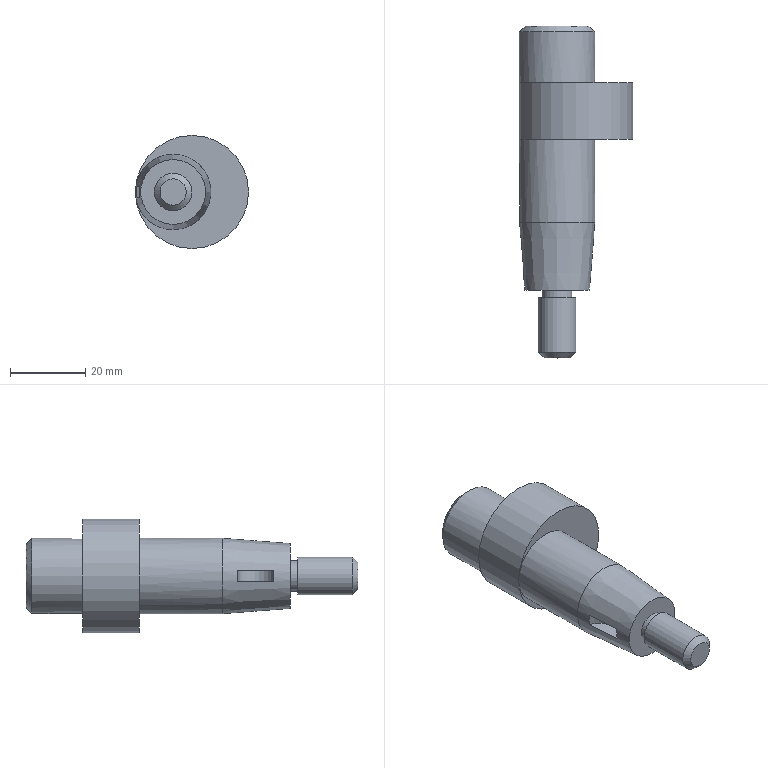Component | NX | ECCENTRIC_SHAFT | 1 solid | 17 faces | box 30 x 88 x 30 mm | volume 28312 mm3 | plane 8 | cylinder 6 | cone 3 | commonest cylinder face diameters 20 x2 10 x2 8 x1 30 x1
STEP:
#1=CARTESIAN_POINT('',(0.,0.,0.));
#2=DIRECTION('',(0.,0.,1.));
#3=DIRECTION('',(1.,0.,0.));
#4=AXIS2_PLACEMENT_3D('',#1,#2,#3);
#5=CARTESIAN_POINT('',(-95.326,-167.11,40.));
#6=VERTEX_POINT('',#5);
#7=CARTESIAN_POINT('',(-95.326,-167.11,50.));
#8=DIRECTION('',(0.,1.,0.));
#9=DIRECTION('',(0.,0.,-1.));
#10=AXIS2_PLACEMENT_3D('',#7,#8,#9);
#11=CIRCLE('',#10,10.);
#12=CARTESIAN_POINT('',(-95.326,-185.11,50.));
#13=DIRECTION('',(0.,1.,0.));
#14=DIRECTION('',(0.,0.,-1.));
#15=AXIS2_PLACEMENT_3D('',#12,#13,#14);
#16=CONICAL_SURFACE('',#15,8.599,0.0777);
#17=CARTESIAN_POINT('',(0.,18.));
#18=DIRECTION('',(1.,0.));
#19=VECTOR('',#18,1.);
#20=LINE('',#17,#19);
#21=(GEOMETRIC_REPRESENTATION_CONTEXT(2)PARAMETRIC_REPRESENTATION_CONTEXT()REPRESENTATION_CONTEXT('',''));
#22=DEFINITIONAL_REPRESENTATION('',(#20),#21);
#23=PCURVE('',#16,#22);
#24=CARTESIAN_POINT('',(-95.326,-203.11,50.));
#25=DIRECTION('',(0.,1.,0.));
#26=DIRECTION('',(0.,0.,-1.));
#27=AXIS2_PLACEMENT_3D('',#24,#25,#26);
#28=CYLINDRICAL_SURFACE('',#27,10.);
#29=CARTESIAN_POINT('',(0.,36.));
#30=DIRECTION('',(1.,0.));
#31=VECTOR('',#30,1.);
#32=LINE('',#29,#31);
#33=(GEOMETRIC_REPRESENTATION_CONTEXT(2)PARAMETRIC_REPRESENTATION_CONTEXT()REPRESENTATION_CONTEXT('',''));
#34=DEFINITIONAL_REPRESENTATION('',(#32),#33);
#35=PCURVE('',#28,#34);
#36=SURFACE_CURVE('',#11,(#23,#35),.PCURVE_S1.);
#37=EDGE_CURVE('',#6,#6,#36,.T.);
#38=ORIENTED_EDGE('',*,*,#37,.F.);
#39=CARTESIAN_POINT('',(-95.326,-185.11,41.401));
#40=VERTEX_POINT('',#39);
#41=CARTESIAN_POINT('',(-95.326,-185.11,41.401));
#42=CARTESIAN_POINT('',(-95.326,-167.11,40.));
#43=B_SPLINE_CURVE_WITH_KNOTS('',1,(#41,#42),.UNSPECIFIED.,.F.,.F.,(2,2),(0.,18.054),.PIECEWISE_BEZIER_KNOTS.);
#44=CARTESIAN_POINT('',(0.,0.));
#45=DIRECTION('',(0.,1.));
#46=VECTOR('',#45,1.);
#47=LINE('',#44,#46);
#48=(GEOMETRIC_REPRESENTATION_CONTEXT(2)PARAMETRIC_REPRESENTATION_CONTEXT()REPRESENTATION_CONTEXT('',''));
#49=DEFINITIONAL_REPRESENTATION('',(#47),#48);
#50=PCURVE('',#16,#49);
#51=CARTESIAN_POINT('',(6.283,0.));
#52=DIRECTION('',(0.,1.));
#53=VECTOR('',#52,1.);
#54=LINE('',#51,#53);
#55=(GEOMETRIC_REPRESENTATION_CONTEXT(2)PARAMETRIC_REPRESENTATION_CONTEXT()REPRESENTATION_CONTEXT('',''));
#56=DEFINITIONAL_REPRESENTATION('',(#54),#55);
#57=PCURVE('',#16,#56);
#58=SEAM_CURVE('',#43,(#50,#57),.PCURVE_S1.);
#59=EDGE_CURVE('',#40,#6,#58,.T.);
#60=ORIENTED_EDGE('',*,*,#59,.F.);
#61=CARTESIAN_POINT('',(-95.326,-185.11,50.));
#62=DIRECTION('',(0.,1.,0.));
#63=DIRECTION('',(0.,0.,-1.));
#64=AXIS2_PLACEMENT_3D('',#61,#62,#63);
#65=CIRCLE('',#64,8.599);
#66=CARTESIAN_POINT('',(0.,0.));
#67=DIRECTION('',(1.,0.));
#68=VECTOR('',#67,1.);
#69=LINE('',#66,#68);
#70=(GEOMETRIC_REPRESENTATION_CONTEXT(2)PARAMETRIC_REPRESENTATION_CONTEXT()REPRESENTATION_CONTEXT('',''));
#71=DEFINITIONAL_REPRESENTATION('',(#69),#70);
#72=PCURVE('',#16,#71);
#73=CARTESIAN_POINT('',(-95.326,-185.11,54.));
#74=DIRECTION('',(0.,1.,0.));
#75=DIRECTION('',(0.,0.,-1.));
#76=AXIS2_PLACEMENT_3D('',#73,#74,#75);
#77=PLANE('',#76);
#78=CARTESIAN_POINT('',(4.,0.));
#79=DIRECTION('',(1.,0.));
#80=AXIS2_PLACEMENT_2D('',#78,#79);
#81=CIRCLE('',#80,8.599);
#82=(GEOMETRIC_REPRESENTATION_CONTEXT(2)PARAMETRIC_REPRESENTATION_CONTEXT()REPRESENTATION_CONTEXT('',''));
#83=DEFINITIONAL_REPRESENTATION('',(#81),#82);
#84=PCURVE('',#77,#83);
#85=SURFACE_CURVE('',#65,(#72,#84),.PCURVE_S1.);
#86=EDGE_CURVE('',#40,#40,#85,.T.);
#87=ORIENTED_EDGE('',*,*,#86,.T.);
#88=ORIENTED_EDGE('',*,*,#59,.T.);
#89=EDGE_LOOP('',(#38,#60,#87,#88));
#90=FACE_BOUND('',#89,.T.);
#91=CARTESIAN_POINT('',(-104.886,-171.267,51.5));
#92=VERTEX_POINT('',#91);
#93=CARTESIAN_POINT('',(-104.142,-180.698,51.5));
#94=VERTEX_POINT('',#93);
#95=CARTESIAN_POINT('',(-104.886,-171.267,51.5));
#96=CARTESIAN_POINT('',(-104.854,-171.674,51.5));
#97=CARTESIAN_POINT('',(-104.822,-172.08,51.5));
#98=CARTESIAN_POINT('',(-104.79,-172.487,51.5));
#99=CARTESIAN_POINT('',(-104.574,-175.224,51.5));
#100=CARTESIAN_POINT('',(-104.358,-177.961,51.5));
#101=CARTESIAN_POINT('',(-104.142,-180.698,51.5));
#102=B_SPLINE_CURVE_WITH_KNOTS('',3,(#95,#96,#97,#98,#99,#100,#101),.UNSPECIFIED.,.F.,.F.,(4,3,4),(0.,0.1293,1.),.UNSPECIFIED.);
#103=CARTESIAN_POINT('',(1.726,13.843));
#104=CARTESIAN_POINT('',(1.739,4.412));
#105=B_SPLINE_CURVE_WITH_KNOTS('',1,(#103,#104),.UNSPECIFIED.,.F.,.F.,(2,2),(0.,1.),.PIECEWISE_BEZIER_KNOTS.);
#106=(GEOMETRIC_REPRESENTATION_CONTEXT(2)PARAMETRIC_REPRESENTATION_CONTEXT()REPRESENTATION_CONTEXT('',''));
#107=DEFINITIONAL_REPRESENTATION('',(#105),#106);
#108=PCURVE('',#16,#107);
#109=CARTESIAN_POINT('',(-106.13,-176.11,51.5));
#110=DIRECTION('',(0.,0.,1.));
#111=DIRECTION('',(-1.,0.,0.));
#112=AXIS2_PLACEMENT_3D('',#109,#110,#111);
#113=PLANE('',#112);
#114=CARTESIAN_POINT('',(-1.244,-4.843));
#115=CARTESIAN_POINT('',(-1.277,-4.436));
#116=CARTESIAN_POINT('',(-1.309,-4.03));
#117=CARTESIAN_POINT('',(-1.341,-3.623));
#118=CARTESIAN_POINT('',(-1.556,-0.8864));
#119=CARTESIAN_POINT('',(-1.772,1.851));
#120=CARTESIAN_POINT('',(-1.988,4.588));
#121=B_SPLINE_CURVE_WITH_KNOTS('',3,(#114,#115,#116,#117,#118,#119,#120),.UNSPECIFIED.,.F.,.F.,(4,3,4),(0.,0.1293,1.),.UNSPECIFIED.);
#122=(GEOMETRIC_REPRESENTATION_CONTEXT(2)PARAMETRIC_REPRESENTATION_CONTEXT()REPRESENTATION_CONTEXT('',''));
#123=DEFINITIONAL_REPRESENTATION('',(#121),#122);
#124=PCURVE('',#113,#123);
#125=SURFACE_CURVE('',#102,(#108,#124),.PCURVE_S1.);
#126=EDGE_CURVE('',#92,#94,#125,.T.);
#127=ORIENTED_EDGE('',*,*,#126,.T.);
#128=CARTESIAN_POINT('',(-104.142,-180.698,48.5));
#129=VERTEX_POINT('',#128);
#130=CARTESIAN_POINT('',(-104.142,-180.698,48.5));
#131=CARTESIAN_POINT('',(-104.306,-180.769,49.496));
#132=CARTESIAN_POINT('',(-104.305,-180.769,50.504));
#133=CARTESIAN_POINT('',(-104.142,-180.698,51.5));
#134=B_SPLINE_CURVE_WITH_KNOTS('',3,(#130,#131,#132,#133),.UNSPECIFIED.,.F.,.F.,(4,4),(0.,1.),.PIECEWISE_BEZIER_KNOTS.);
#135=CARTESIAN_POINT('',(1.402,4.412));
#136=CARTESIAN_POINT('',(1.407,4.409));
#137=CARTESIAN_POINT('',(1.418,4.403));
#138=CARTESIAN_POINT('',(1.433,4.395));
#139=CARTESIAN_POINT('',(1.448,4.387));
#140=CARTESIAN_POINT('',(1.464,4.381));
#141=CARTESIAN_POINT('',(1.479,4.375));
#142=CARTESIAN_POINT('',(1.494,4.37));
#143=CARTESIAN_POINT('',(1.51,4.366));
#144=CARTESIAN_POINT('',(1.525,4.363));
#145=CARTESIAN_POINT('',(1.54,4.361));
#146=CARTESIAN_POINT('',(1.556,4.359));
#147=CARTESIAN_POINT('',(1.571,4.359));
#148=CARTESIAN_POINT('',(1.586,4.359));
#149=CARTESIAN_POINT('',(1.601,4.361));
#150=CARTESIAN_POINT('',(1.617,4.363));
#151=CARTESIAN_POINT('',(1.632,4.366));
#152=CARTESIAN_POINT('',(1.647,4.37));
#153=CARTESIAN_POINT('',(1.663,4.375));
#154=CARTESIAN_POINT('',(1.678,4.381));
#155=CARTESIAN_POINT('',(1.693,4.387));
#156=CARTESIAN_POINT('',(1.709,4.395));
#157=CARTESIAN_POINT('',(1.724,4.403));
#158=CARTESIAN_POINT('',(1.734,4.409));
#159=CARTESIAN_POINT('',(1.739,4.412));
#160=B_SPLINE_CURVE_WITH_KNOTS('',3,(#135,#136,#137,#138,#139,#140,#141,#142,#143,#144,#145,#146,#147,#148,#149,#150,#151,#152,#153,#154,#155,#156,#157,#158,#159),.UNSPECIFIED.,.F.,.F.,(4,1,1,1,1,1,1,1,1,1,1,1,1,1,1,1,1,1,1,1,1,1,4),(0.,0.04545,0.09091,0.1364,0.1818,0.2273,0.2727,0.3182,0.3636,0.4091,0.4545,0.5,0.5455,0.5909,0.6364,0.6818,0.7273,0.7727,0.8182,0.8636,0.9091,0.9545,1.),.QUASI_UNIFORM_KNOTS.);
#161=(GEOMETRIC_REPRESENTATION_CONTEXT(2)PARAMETRIC_REPRESENTATION_CONTEXT()REPRESENTATION_CONTEXT('',''));
#162=DEFINITIONAL_REPRESENTATION('',(#160),#161);
#163=PCURVE('',#16,#162);
#164=CARTESIAN_POINT('',(-106.13,-176.11,51.5));
#165=DIRECTION('',(0.,0.,-1.));
#166=DIRECTION('',(1.,0.,0.));
#167=AXIS2_PLACEMENT_3D('',#164,#165,#166);
#168=CYLINDRICAL_SURFACE('',#167,5.);
#169=CARTESIAN_POINT('',(7.445,3.));
#170=CARTESIAN_POINT('',(7.447,2.955));
#171=CARTESIAN_POINT('',(7.45,2.864));
#172=CARTESIAN_POINT('',(7.454,2.728));
#173=CARTESIAN_POINT('',(7.458,2.592));
#174=CARTESIAN_POINT('',(7.461,2.456));
#175=CARTESIAN_POINT('',(7.464,2.319));
#176=CARTESIAN_POINT('',(7.466,2.183));
#177=CARTESIAN_POINT('',(7.468,2.046));
#178=CARTESIAN_POINT('',(7.47,1.91));
#179=CARTESIAN_POINT('',(7.471,1.773));
#180=CARTESIAN_POINT('',(7.472,1.637));
#181=CARTESIAN_POINT('',(7.472,1.5));
#182=CARTESIAN_POINT('',(7.472,1.363));
#183=CARTESIAN_POINT('',(7.471,1.227));
#184=CARTESIAN_POINT('',(7.47,1.09));
#185=CARTESIAN_POINT('',(7.468,0.9535));
#186=CARTESIAN_POINT('',(7.466,0.817));
#187=CARTESIAN_POINT('',(7.464,0.6806));
#188=CARTESIAN_POINT('',(7.461,0.5442));
#189=CARTESIAN_POINT('',(7.458,0.408));
#190=CARTESIAN_POINT('',(7.454,0.2718));
#191=CARTESIAN_POINT('',(7.45,0.1358));
#192=CARTESIAN_POINT('',(7.447,0.04526));
#193=CARTESIAN_POINT('',(7.445,0.));
#194=B_SPLINE_CURVE_WITH_KNOTS('',3,(#169,#170,#171,#172,#173,#174,#175,#176,#177,#178,#179,#180,#181,#182,#183,#184,#185,#186,#187,#188,#189,#190,#191,#192,#193),.UNSPECIFIED.,.F.,.F.,(4,1,1,1,1,1,1,1,1,1,1,1,1,1,1,1,1,1,1,1,1,1,4),(0.,0.04545,0.09091,0.1364,0.1818,0.2273,0.2727,0.3182,0.3636,0.4091,0.4545,0.5,0.5455,0.5909,0.6364,0.6818,0.7273,0.7727,0.8182,0.8636,0.9091,0.9545,1.),.QUASI_UNIFORM_KNOTS.);
#195=(GEOMETRIC_REPRESENTATION_CONTEXT(2)PARAMETRIC_REPRESENTATION_CONTEXT()REPRESENTATION_CONTEXT('',''));
#196=DEFINITIONAL_REPRESENTATION('',(#194),#195);
#197=PCURVE('',#168,#196);
#198=SURFACE_CURVE('',#134,(#163,#197),.PCURVE_S1.);
#199=EDGE_CURVE('',#129,#94,#198,.T.);
#200=ORIENTED_EDGE('',*,*,#199,.F.);
#201=CARTESIAN_POINT('',(-104.886,-171.267,48.5));
#202=VERTEX_POINT('',#201);
#203=CARTESIAN_POINT('',(-104.886,-171.267,48.5));
#204=CARTESIAN_POINT('',(-104.854,-171.674,48.5));
#205=CARTESIAN_POINT('',(-104.822,-172.08,48.5));
#206=CARTESIAN_POINT('',(-104.79,-172.487,48.5));
#207=CARTESIAN_POINT('',(-104.574,-175.224,48.5));
#208=CARTESIAN_POINT('',(-104.358,-177.961,48.5));
#209=CARTESIAN_POINT('',(-104.142,-180.698,48.5));
#210=B_SPLINE_CURVE_WITH_KNOTS('',3,(#203,#204,#205,#206,#207,#208,#209),.UNSPECIFIED.,.F.,.F.,(4,3,4),(0.,0.1293,1.),.UNSPECIFIED.);
#211=CARTESIAN_POINT('',(1.415,13.843));
#212=CARTESIAN_POINT('',(1.402,4.412));
#213=B_SPLINE_CURVE_WITH_KNOTS('',1,(#211,#212),.UNSPECIFIED.,.F.,.F.,(2,2),(0.,1.),.PIECEWISE_BEZIER_KNOTS.);
#214=(GEOMETRIC_REPRESENTATION_CONTEXT(2)PARAMETRIC_REPRESENTATION_CONTEXT()REPRESENTATION_CONTEXT('',''));
#215=DEFINITIONAL_REPRESENTATION('',(#213),#214);
#216=PCURVE('',#16,#215);
#217=CARTESIAN_POINT('',(-106.13,-176.11,48.5));
#218=DIRECTION('',(0.,0.,1.));
#219=DIRECTION('',(-1.,0.,0.));
#220=AXIS2_PLACEMENT_3D('',#217,#218,#219);
#221=PLANE('',#220);
#222=CARTESIAN_POINT('',(-1.244,-4.843));
#223=CARTESIAN_POINT('',(-1.277,-4.436));
#224=CARTESIAN_POINT('',(-1.309,-4.03));
#225=CARTESIAN_POINT('',(-1.341,-3.623));
#226=CARTESIAN_POINT('',(-1.556,-0.8864));
#227=CARTESIAN_POINT('',(-1.772,1.851));
#228=CARTESIAN_POINT('',(-1.988,4.588));
#229=B_SPLINE_CURVE_WITH_KNOTS('',3,(#222,#223,#224,#225,#226,#227,#228),.UNSPECIFIED.,.F.,.F.,(4,3,4),(0.,0.1293,1.),.UNSPECIFIED.);
#230=(GEOMETRIC_REPRESENTATION_CONTEXT(2)PARAMETRIC_REPRESENTATION_CONTEXT()REPRESENTATION_CONTEXT('',''));
#231=DEFINITIONAL_REPRESENTATION('',(#229),#230);
#232=PCURVE('',#221,#231);
#233=SURFACE_CURVE('',#210,(#216,#232),.PCURVE_S1.);
#234=EDGE_CURVE('',#202,#129,#233,.T.);
#235=ORIENTED_EDGE('',*,*,#234,.F.);
#236=CARTESIAN_POINT('',(-104.886,-171.267,51.5));
#237=CARTESIAN_POINT('',(-105.046,-171.226,50.5));
#238=CARTESIAN_POINT('',(-105.046,-171.226,49.5));
#239=CARTESIAN_POINT('',(-104.886,-171.267,48.5));
#240=B_SPLINE_CURVE_WITH_KNOTS('',3,(#236,#237,#238,#239),.UNSPECIFIED.,.F.,.F.,(4,4),(0.,1.),.PIECEWISE_BEZIER_KNOTS.);
#241=CARTESIAN_POINT('',(1.726,13.843));
#242=CARTESIAN_POINT('',(1.415,13.843));
#243=B_SPLINE_CURVE_WITH_KNOTS('',1,(#241,#242),.UNSPECIFIED.,.F.,.F.,(2,2),(0.,1.),.PIECEWISE_BEZIER_KNOTS.);
#244=(GEOMETRIC_REPRESENTATION_CONTEXT(2)PARAMETRIC_REPRESENTATION_CONTEXT()REPRESENTATION_CONTEXT('',''));
#245=DEFINITIONAL_REPRESENTATION('',(#243),#244);
#246=PCURVE('',#16,#245);
#247=CARTESIAN_POINT('',(4.964,0.));
#248=CARTESIAN_POINT('',(4.962,0.04545));
#249=CARTESIAN_POINT('',(4.96,0.1364));
#250=CARTESIAN_POINT('',(4.956,0.2727));
#251=CARTESIAN_POINT('',(4.952,0.4091));
#252=CARTESIAN_POINT('',(4.949,0.5455));
#253=CARTESIAN_POINT('',(4.946,0.6818));
#254=CARTESIAN_POINT('',(4.944,0.8182));
#255=CARTESIAN_POINT('',(4.942,0.9545));
#256=CARTESIAN_POINT('',(4.941,1.091));
#257=CARTESIAN_POINT('',(4.94,1.227));
#258=CARTESIAN_POINT('',(4.939,1.364));
#259=CARTESIAN_POINT('',(4.939,1.5));
#260=CARTESIAN_POINT('',(4.939,1.636));
#261=CARTESIAN_POINT('',(4.94,1.773));
#262=CARTESIAN_POINT('',(4.941,1.909));
#263=CARTESIAN_POINT('',(4.942,2.045));
#264=CARTESIAN_POINT('',(4.944,2.182));
#265=CARTESIAN_POINT('',(4.946,2.318));
#266=CARTESIAN_POINT('',(4.949,2.455));
#267=CARTESIAN_POINT('',(4.952,2.591));
#268=CARTESIAN_POINT('',(4.956,2.727));
#269=CARTESIAN_POINT('',(4.96,2.864));
#270=CARTESIAN_POINT('',(4.962,2.955));
#271=CARTESIAN_POINT('',(4.964,3.));
#272=B_SPLINE_CURVE_WITH_KNOTS('',3,(#247,#248,#249,#250,#251,#252,#253,#254,#255,#256,#257,#258,#259,#260,#261,#262,#263,#264,#265,#266,#267,#268,#269,#270,#271),.UNSPECIFIED.,.F.,.F.,(4,1,1,1,1,1,1,1,1,1,1,1,1,1,1,1,1,1,1,1,1,1,4),(0.,0.04545,0.09091,0.1364,0.1818,0.2273,0.2727,0.3182,0.3636,0.4091,0.4545,0.5,0.5455,0.5909,0.6364,0.6818,0.7273,0.7727,0.8182,0.8636,0.9091,0.9545,1.),.QUASI_UNIFORM_KNOTS.);
#273=(GEOMETRIC_REPRESENTATION_CONTEXT(2)PARAMETRIC_REPRESENTATION_CONTEXT()REPRESENTATION_CONTEXT('',''));
#274=DEFINITIONAL_REPRESENTATION('',(#272),#273);
#275=PCURVE('',#168,#274);
#276=SURFACE_CURVE('',#240,(#246,#275),.PCURVE_S1.);
#277=EDGE_CURVE('',#92,#202,#276,.T.);
#278=ORIENTED_EDGE('',*,*,#277,.F.);
#279=EDGE_LOOP('',(#127,#200,#235,#278));
#280=FACE_BOUND('',#279,.T.);
#281=ADVANCED_FACE('',(#90,#280),#16,.T.);
#282=ORIENTED_EDGE('',*,*,#37,.T.);
#283=CARTESIAN_POINT('',(-95.326,-145.11,40.));
#284=VERTEX_POINT('',#283);
#285=CARTESIAN_POINT('',(-95.326,-167.11,40.));
#286=CARTESIAN_POINT('',(-95.326,-145.11,40.));
#287=B_SPLINE_CURVE_WITH_KNOTS('',1,(#285,#286),.UNSPECIFIED.,.F.,.F.,(2,2),(36.,58.),.PIECEWISE_BEZIER_KNOTS.);
#288=CARTESIAN_POINT('',(6.283,0.));
#289=DIRECTION('',(0.,1.));
#290=VECTOR('',#289,1.);
#291=LINE('',#288,#290);
#292=(GEOMETRIC_REPRESENTATION_CONTEXT(2)PARAMETRIC_REPRESENTATION_CONTEXT()REPRESENTATION_CONTEXT('',''));
#293=DEFINITIONAL_REPRESENTATION('',(#291),#292);
#294=PCURVE('',#28,#293);
#295=CARTESIAN_POINT('',(0.,0.));
#296=DIRECTION('',(0.,1.));
#297=VECTOR('',#296,1.);
#298=LINE('',#295,#297);
#299=(GEOMETRIC_REPRESENTATION_CONTEXT(2)PARAMETRIC_REPRESENTATION_CONTEXT()REPRESENTATION_CONTEXT('',''));
#300=DEFINITIONAL_REPRESENTATION('',(#298),#299);
#301=PCURVE('',#28,#300);
#302=SEAM_CURVE('',#287,(#294,#301),.PCURVE_S1.);
#303=EDGE_CURVE('',#6,#284,#302,.T.);
#304=ORIENTED_EDGE('',*,*,#303,.T.);
#305=CARTESIAN_POINT('',(-105.326,-145.11,50.));
#306=VERTEX_POINT('',#305);
#307=CARTESIAN_POINT('',(-95.326,-145.11,50.));
#308=DIRECTION('',(0.,1.,0.));
#309=DIRECTION('',(0.,0.,-1.));
#310=AXIS2_PLACEMENT_3D('',#307,#308,#309);
#311=CIRCLE('',#310,10.);
#312=CARTESIAN_POINT('',(0.,58.));
#313=DIRECTION('',(1.,0.));
#314=VECTOR('',#313,1.);
#315=LINE('',#312,#314);
#316=(GEOMETRIC_REPRESENTATION_CONTEXT(2)PARAMETRIC_REPRESENTATION_CONTEXT()REPRESENTATION_CONTEXT('',''));
#317=DEFINITIONAL_REPRESENTATION('',(#315),#316);
#318=PCURVE('',#28,#317);
#319=CARTESIAN_POINT('',(-90.326,-145.11,50.));
#320=DIRECTION('',(0.,1.,0.));
#321=DIRECTION('',(0.,0.,-1.));
#322=AXIS2_PLACEMENT_3D('',#319,#320,#321);
#323=PLANE('',#322);
#324=CARTESIAN_POINT('',(0.,5.));
#325=DIRECTION('',(1.,0.));
#326=AXIS2_PLACEMENT_2D('',#324,#325);
#327=CIRCLE('',#326,10.);
#328=(GEOMETRIC_REPRESENTATION_CONTEXT(2)PARAMETRIC_REPRESENTATION_CONTEXT()REPRESENTATION_CONTEXT('',''));
#329=DEFINITIONAL_REPRESENTATION('',(#327),#328);
#330=PCURVE('',#323,#329);
#331=SURFACE_CURVE('',#311,(#318,#330),.PCURVE_S1.);
#332=EDGE_CURVE('',#306,#284,#331,.T.);
#333=ORIENTED_EDGE('',*,*,#332,.F.);
#334=CARTESIAN_POINT('',(-95.326,-145.11,50.));
#335=DIRECTION('',(0.,1.,0.));
#336=DIRECTION('',(0.,0.,-1.));
#337=AXIS2_PLACEMENT_3D('',#334,#335,#336);
#338=CIRCLE('',#337,10.);
#339=CARTESIAN_POINT('',(-6.283,58.));
#340=DIRECTION('',(1.,0.));
#341=VECTOR('',#340,1.);
#342=LINE('',#339,#341);
#343=(GEOMETRIC_REPRESENTATION_CONTEXT(2)PARAMETRIC_REPRESENTATION_CONTEXT()REPRESENTATION_CONTEXT('',''));
#344=DEFINITIONAL_REPRESENTATION('',(#342),#343);
#345=PCURVE('',#28,#344);
#346=CARTESIAN_POINT('',(0.,5.));
#347=DIRECTION('',(1.,0.));
#348=AXIS2_PLACEMENT_2D('',#346,#347);
#349=CIRCLE('',#348,10.);
#350=(GEOMETRIC_REPRESENTATION_CONTEXT(2)PARAMETRIC_REPRESENTATION_CONTEXT()REPRESENTATION_CONTEXT('',''));
#351=DEFINITIONAL_REPRESENTATION('',(#349),#350);
#352=PCURVE('',#323,#351);
#353=SURFACE_CURVE('',#338,(#345,#352),.PCURVE_S1.);
#354=EDGE_CURVE('',#284,#306,#353,.T.);
#355=ORIENTED_EDGE('',*,*,#354,.F.);
#356=ORIENTED_EDGE('',*,*,#303,.F.);
#357=EDGE_LOOP('',(#282,#304,#333,#355,#356));
#358=FACE_BOUND('',#357,.T.);
#359=ADVANCED_FACE('',(#358),#28,.T.);
#360=CARTESIAN_POINT('',(-95.326,-203.11,46.5));
#361=VERTEX_POINT('',#360);
#362=CARTESIAN_POINT('',(-95.326,-203.11,50.));
#363=DIRECTION('',(0.,-1.,0.));
#364=DIRECTION('',(0.,0.,-1.));
#365=AXIS2_PLACEMENT_3D('',#362,#363,#364);
#366=CIRCLE('',#365,3.5);
#367=CARTESIAN_POINT('',(-95.326,-203.11,50.));
#368=DIRECTION('',(0.,1.,0.));
#369=DIRECTION('',(0.,0.,-1.));
#370=AXIS2_PLACEMENT_3D('',#367,#368,#369);
#371=PLANE('',#370);
#372=CARTESIAN_POINT('',(3.5,0.));
#373=CARTESIAN_POINT('',(3.5,-6.062));
#374=CARTESIAN_POINT('',(-1.75,-3.031));
#375=CARTESIAN_POINT('',(-7.,-0.));
#376=CARTESIAN_POINT('',(-1.75,3.031));
#377=CARTESIAN_POINT('',(3.5,6.062));
#378=CARTESIAN_POINT('',(3.5,0.));
#379=(BOUNDED_CURVE()B_SPLINE_CURVE(2,(#372,#373,#374,#375,#376,#377,#378),.UNSPECIFIED.,.T.,.F.)B_SPLINE_CURVE_WITH_KNOTS((1,2,2,2,2,1),(-2.094,0.,2.094,4.189,6.283,8.378),.UNSPECIFIED.)CURVE()GEOMETRIC_REPRESENTATION_ITEM()RATIONAL_B_SPLINE_CURVE((1.,0.5,1.,0.5,1.,0.5,1.))REPRESENTATION_ITEM(''));
#380=(GEOMETRIC_REPRESENTATION_CONTEXT(2)PARAMETRIC_REPRESENTATION_CONTEXT()REPRESENTATION_CONTEXT('',''));
#381=DEFINITIONAL_REPRESENTATION('',(#379),#380);
#382=PCURVE('',#371,#381);
#383=CARTESIAN_POINT('',(-95.326,-201.61,50.));
#384=DIRECTION('',(0.,1.,0.));
#385=DIRECTION('',(0.,0.,-1.));
#386=AXIS2_PLACEMENT_3D('',#383,#384,#385);
#387=CONICAL_SURFACE('',#386,5.,0.7854);
#388=CARTESIAN_POINT('',(6.283,-1.5));
#389=DIRECTION('',(-1.,0.));
#390=VECTOR('',#389,1.);
#391=LINE('',#388,#390);
#392=(GEOMETRIC_REPRESENTATION_CONTEXT(2)PARAMETRIC_REPRESENTATION_CONTEXT()REPRESENTATION_CONTEXT('',''));
#393=DEFINITIONAL_REPRESENTATION('',(#391),#392);
#394=PCURVE('',#387,#393);
#395=SURFACE_CURVE('',#366,(#382,#394),.PCURVE_S1.);
#396=EDGE_CURVE('',#361,#361,#395,.T.);
#397=ORIENTED_EDGE('',*,*,#396,.T.);
#398=EDGE_LOOP('',(#397));
#399=FACE_BOUND('',#398,.T.);
#400=ADVANCED_FACE('',(#399),#371,.F.);
#401=CARTESIAN_POINT('',(-95.326,-201.61,45.));
#402=VERTEX_POINT('',#401);
#403=CARTESIAN_POINT('',(-95.326,-201.61,50.));
#404=DIRECTION('',(0.,1.,0.));
#405=DIRECTION('',(0.,0.,-1.));
#406=AXIS2_PLACEMENT_3D('',#403,#404,#405);
#407=CIRCLE('',#406,5.);
#408=CARTESIAN_POINT('',(-95.326,-203.11,50.));
#409=DIRECTION('',(0.,1.,0.));
#410=DIRECTION('',(0.,0.,-1.));
#411=AXIS2_PLACEMENT_3D('',#408,#409,#410);
#412=CYLINDRICAL_SURFACE('',#411,5.);
#413=CARTESIAN_POINT('',(0.,1.5));
#414=DIRECTION('',(1.,0.));
#415=VECTOR('',#414,1.);
#416=LINE('',#413,#415);
#417=(GEOMETRIC_REPRESENTATION_CONTEXT(2)PARAMETRIC_REPRESENTATION_CONTEXT()REPRESENTATION_CONTEXT('',''));
#418=DEFINITIONAL_REPRESENTATION('',(#416),#417);
#419=PCURVE('',#412,#418);
#420=CARTESIAN_POINT('',(0.,0.));
#421=DIRECTION('',(1.,0.));
#422=VECTOR('',#421,1.);
#423=LINE('',#420,#422);
#424=(GEOMETRIC_REPRESENTATION_CONTEXT(2)PARAMETRIC_REPRESENTATION_CONTEXT()REPRESENTATION_CONTEXT('',''));
#425=DEFINITIONAL_REPRESENTATION('',(#423),#424);
#426=PCURVE('',#387,#425);
#427=SURFACE_CURVE('',#407,(#419,#426),.PCURVE_S1.);
#428=EDGE_CURVE('',#402,#402,#427,.T.);
#429=ORIENTED_EDGE('',*,*,#428,.T.);
#430=CARTESIAN_POINT('',(-95.326,-187.11,45.));
#431=VERTEX_POINT('',#430);
#432=CARTESIAN_POINT('',(-95.326,-201.61,45.));
#433=CARTESIAN_POINT('',(-95.326,-187.11,45.));
#434=B_SPLINE_CURVE_WITH_KNOTS('',1,(#432,#433),.UNSPECIFIED.,.F.,.F.,(2,2),(1.5,16.),.PIECEWISE_BEZIER_KNOTS.);
#435=CARTESIAN_POINT('',(6.283,0.));
#436=DIRECTION('',(0.,1.));
#437=VECTOR('',#436,1.);
#438=LINE('',#435,#437);
#439=(GEOMETRIC_REPRESENTATION_CONTEXT(2)PARAMETRIC_REPRESENTATION_CONTEXT()REPRESENTATION_CONTEXT('',''));
#440=DEFINITIONAL_REPRESENTATION('',(#438),#439);
#441=PCURVE('',#412,#440);
#442=CARTESIAN_POINT('',(0.,0.));
#443=DIRECTION('',(0.,1.));
#444=VECTOR('',#443,1.);
#445=LINE('',#442,#444);
#446=(GEOMETRIC_REPRESENTATION_CONTEXT(2)PARAMETRIC_REPRESENTATION_CONTEXT()REPRESENTATION_CONTEXT('',''));
#447=DEFINITIONAL_REPRESENTATION('',(#445),#446);
#448=PCURVE('',#412,#447);
#449=SEAM_CURVE('',#434,(#441,#448),.PCURVE_S1.);
#450=EDGE_CURVE('',#402,#431,#449,.T.);
#451=ORIENTED_EDGE('',*,*,#450,.T.);
#452=CARTESIAN_POINT('',(-95.326,-187.11,50.));
#453=DIRECTION('',(0.,1.,0.));
#454=DIRECTION('',(0.,0.,-1.));
#455=AXIS2_PLACEMENT_3D('',#452,#453,#454);
#456=CIRCLE('',#455,5.);
#457=CARTESIAN_POINT('',(0.,16.));
#458=DIRECTION('',(1.,0.));
#459=VECTOR('',#458,1.);
#460=LINE('',#457,#459);
#461=(GEOMETRIC_REPRESENTATION_CONTEXT(2)PARAMETRIC_REPRESENTATION_CONTEXT()REPRESENTATION_CONTEXT('',''));
#462=DEFINITIONAL_REPRESENTATION('',(#460),#461);
#463=PCURVE('',#412,#462);
#464=CARTESIAN_POINT('',(-95.326,-187.11,55.));
#465=DIRECTION('',(0.,-1.,0.));
#466=DIRECTION('',(0.,0.,1.));
#467=AXIS2_PLACEMENT_3D('',#464,#465,#466);
#468=PLANE('',#467);
#469=CARTESIAN_POINT('',(-10.,0.));
#470=CARTESIAN_POINT('',(-10.,8.66));
#471=CARTESIAN_POINT('',(-2.5,4.33));
#472=CARTESIAN_POINT('',(5.,0.));
#473=CARTESIAN_POINT('',(-2.5,-4.33));
#474=CARTESIAN_POINT('',(-10.,-8.66));
#475=CARTESIAN_POINT('',(-10.,0.));
#476=(BOUNDED_CURVE()B_SPLINE_CURVE(2,(#469,#470,#471,#472,#473,#474,#475),.UNSPECIFIED.,.T.,.F.)B_SPLINE_CURVE_WITH_KNOTS((1,2,2,2,2,1),(-2.094,0.,2.094,4.189,6.283,8.378),.UNSPECIFIED.)CURVE()GEOMETRIC_REPRESENTATION_ITEM()RATIONAL_B_SPLINE_CURVE((1.,0.5,1.,0.5,1.,0.5,1.))REPRESENTATION_ITEM(''));
#477=(GEOMETRIC_REPRESENTATION_CONTEXT(2)PARAMETRIC_REPRESENTATION_CONTEXT()REPRESENTATION_CONTEXT('',''));
#478=DEFINITIONAL_REPRESENTATION('',(#476),#477);
#479=PCURVE('',#468,#478);
#480=SURFACE_CURVE('',#456,(#463,#479),.PCURVE_S1.);
#481=EDGE_CURVE('',#431,#431,#480,.T.);
#482=ORIENTED_EDGE('',*,*,#481,.F.);
#483=ORIENTED_EDGE('',*,*,#450,.F.);
#484=EDGE_LOOP('',(#429,#451,#482,#483));
#485=FACE_BOUND('',#484,.T.);
#486=ADVANCED_FACE('',(#485),#412,.T.);
#487=CARTESIAN_POINT('',(-95.326,-187.11,46.));
#488=VERTEX_POINT('',#487);
#489=CARTESIAN_POINT('',(-95.326,-187.11,50.));
#490=DIRECTION('',(0.,1.,0.));
#491=DIRECTION('',(0.,0.,-1.));
#492=AXIS2_PLACEMENT_3D('',#489,#490,#491);
#493=CIRCLE('',#492,4.);
#494=CARTESIAN_POINT('',(-9.,0.));
#495=CARTESIAN_POINT('',(-9.,6.928));
#496=CARTESIAN_POINT('',(-3.,3.464));
#497=CARTESIAN_POINT('',(3.,0.));
#498=CARTESIAN_POINT('',(-3.,-3.464));
#499=CARTESIAN_POINT('',(-9.,-6.928));
#500=CARTESIAN_POINT('',(-9.,0.));
#501=(BOUNDED_CURVE()B_SPLINE_CURVE(2,(#494,#495,#496,#497,#498,#499,#500),.UNSPECIFIED.,.T.,.F.)B_SPLINE_CURVE_WITH_KNOTS((1,2,2,2,2,1),(-2.094,0.,2.094,4.189,6.283,8.378),.UNSPECIFIED.)CURVE()GEOMETRIC_REPRESENTATION_ITEM()RATIONAL_B_SPLINE_CURVE((1.,0.5,1.,0.5,1.,0.5,1.))REPRESENTATION_ITEM(''));
#502=(GEOMETRIC_REPRESENTATION_CONTEXT(2)PARAMETRIC_REPRESENTATION_CONTEXT()REPRESENTATION_CONTEXT('',''));
#503=DEFINITIONAL_REPRESENTATION('',(#501),#502);
#504=PCURVE('',#468,#503);
#505=CARTESIAN_POINT('',(-95.326,-203.11,50.));
#506=DIRECTION('',(0.,1.,0.));
#507=DIRECTION('',(0.,0.,-1.));
#508=AXIS2_PLACEMENT_3D('',#505,#506,#507);
#509=CYLINDRICAL_SURFACE('',#508,4.);
#510=CARTESIAN_POINT('',(0.,16.));
#511=DIRECTION('',(1.,0.));
#512=VECTOR('',#511,1.);
#513=LINE('',#510,#512);
#514=(GEOMETRIC_REPRESENTATION_CONTEXT(2)PARAMETRIC_REPRESENTATION_CONTEXT()REPRESENTATION_CONTEXT('',''));
#515=DEFINITIONAL_REPRESENTATION('',(#513),#514);
#516=PCURVE('',#509,#515);
#517=SURFACE_CURVE('',#493,(#504,#516),.PCURVE_S1.);
#518=EDGE_CURVE('',#488,#488,#517,.T.);
#519=ORIENTED_EDGE('',*,*,#518,.F.);
#520=EDGE_LOOP('',(#519));
#521=FACE_BOUND('',#520,.T.);
#522=ORIENTED_EDGE('',*,*,#481,.T.);
#523=EDGE_LOOP('',(#522));
#524=FACE_BOUND('',#523,.T.);
#525=ADVANCED_FACE('',(#521,#524),#468,.F.);
#526=CARTESIAN_POINT('',(-95.326,-185.11,46.));
#527=VERTEX_POINT('',#526);
#528=CARTESIAN_POINT('',(-95.326,-185.11,50.));
#529=DIRECTION('',(0.,1.,0.));
#530=DIRECTION('',(0.,0.,-1.));
#531=AXIS2_PLACEMENT_3D('',#528,#529,#530);
#532=CIRCLE('',#531,4.);
#533=CARTESIAN_POINT('',(0.,18.));
#534=DIRECTION('',(1.,0.));
#535=VECTOR('',#534,1.);
#536=LINE('',#533,#535);
#537=(GEOMETRIC_REPRESENTATION_CONTEXT(2)PARAMETRIC_REPRESENTATION_CONTEXT()REPRESENTATION_CONTEXT('',''));
#538=DEFINITIONAL_REPRESENTATION('',(#536),#537);
#539=PCURVE('',#509,#538);
#540=CARTESIAN_POINT('',(4.,0.));
#541=DIRECTION('',(1.,0.));
#542=AXIS2_PLACEMENT_2D('',#540,#541);
#543=CIRCLE('',#542,4.);
#544=(GEOMETRIC_REPRESENTATION_CONTEXT(2)PARAMETRIC_REPRESENTATION_CONTEXT()REPRESENTATION_CONTEXT('',''));
#545=DEFINITIONAL_REPRESENTATION('',(#543),#544);
#546=PCURVE('',#77,#545);
#547=SURFACE_CURVE('',#532,(#539,#546),.PCURVE_S1.);
#548=EDGE_CURVE('',#527,#527,#547,.T.);
#549=ORIENTED_EDGE('',*,*,#548,.F.);
#550=CARTESIAN_POINT('',(-95.326,-187.11,46.));
#551=CARTESIAN_POINT('',(-95.326,-185.11,46.));
#552=B_SPLINE_CURVE_WITH_KNOTS('',1,(#550,#551),.UNSPECIFIED.,.F.,.F.,(2,2),(16.,18.),.PIECEWISE_BEZIER_KNOTS.);
#553=CARTESIAN_POINT('',(0.,0.));
#554=DIRECTION('',(0.,1.));
#555=VECTOR('',#554,1.);
#556=LINE('',#553,#555);
#557=(GEOMETRIC_REPRESENTATION_CONTEXT(2)PARAMETRIC_REPRESENTATION_CONTEXT()REPRESENTATION_CONTEXT('',''));
#558=DEFINITIONAL_REPRESENTATION('',(#556),#557);
#559=PCURVE('',#509,#558);
#560=CARTESIAN_POINT('',(6.283,0.));
#561=DIRECTION('',(0.,1.));
#562=VECTOR('',#561,1.);
#563=LINE('',#560,#562);
#564=(GEOMETRIC_REPRESENTATION_CONTEXT(2)PARAMETRIC_REPRESENTATION_CONTEXT()REPRESENTATION_CONTEXT('',''));
#565=DEFINITIONAL_REPRESENTATION('',(#563),#564);
#566=PCURVE('',#509,#565);
#567=SEAM_CURVE('',#552,(#559,#566),.PCURVE_S1.);
#568=EDGE_CURVE('',#488,#527,#567,.T.);
#569=ORIENTED_EDGE('',*,*,#568,.F.);
#570=ORIENTED_EDGE('',*,*,#518,.T.);
#571=ORIENTED_EDGE('',*,*,#568,.T.);
#572=EDGE_LOOP('',(#549,#569,#570,#571));
#573=FACE_BOUND('',#572,.T.);
#574=ADVANCED_FACE('',(#573),#509,.T.);
#575=ORIENTED_EDGE('',*,*,#86,.F.);
#576=EDGE_LOOP('',(#575));
#577=FACE_BOUND('',#576,.T.);
#578=ORIENTED_EDGE('',*,*,#548,.T.);
#579=EDGE_LOOP('',(#578));
#580=FACE_BOUND('',#579,.T.);
#581=ADVANCED_FACE('',(#577,#580),#77,.F.);
#582=CARTESIAN_POINT('',(-105.326,-130.11,50.));
#583=VERTEX_POINT('',#582);
#584=CARTESIAN_POINT('',(-90.326,-130.11,50.));
#585=DIRECTION('',(0.,1.,0.));
#586=DIRECTION('',(-1.,0.,0.));
#587=AXIS2_PLACEMENT_3D('',#584,#585,#586);
#588=CIRCLE('',#587,15.);
#589=CARTESIAN_POINT('',(-90.326,-145.11,50.));
#590=DIRECTION('',(0.,1.,0.));
#591=DIRECTION('',(0.,0.,-1.));
#592=AXIS2_PLACEMENT_3D('',#589,#590,#591);
#593=CYLINDRICAL_SURFACE('',#592,15.);
#594=CARTESIAN_POINT('',(1.571,15.));
#595=DIRECTION('',(1.,0.));
#596=VECTOR('',#595,1.);
#597=LINE('',#594,#596);
#598=(GEOMETRIC_REPRESENTATION_CONTEXT(2)PARAMETRIC_REPRESENTATION_CONTEXT()REPRESENTATION_CONTEXT('',''));
#599=DEFINITIONAL_REPRESENTATION('',(#597),#598);
#600=PCURVE('',#593,#599);
#601=CARTESIAN_POINT('',(-90.326,-130.11,50.));
#602=DIRECTION('',(0.,1.,0.));
#603=DIRECTION('',(0.,0.,-1.));
#604=AXIS2_PLACEMENT_3D('',#601,#602,#603);
#605=PLANE('',#604);
#606=CARTESIAN_POINT('',(0.,0.));
#607=DIRECTION('',(0.,1.));
#608=AXIS2_PLACEMENT_2D('',#606,#607);
#609=CIRCLE('',#608,15.);
#610=(GEOMETRIC_REPRESENTATION_CONTEXT(2)PARAMETRIC_REPRESENTATION_CONTEXT()REPRESENTATION_CONTEXT('',''));
#611=DEFINITIONAL_REPRESENTATION('',(#609),#610);
#612=PCURVE('',#605,#611);
#613=SURFACE_CURVE('',#588,(#600,#612),.PCURVE_S1.);
#614=EDGE_CURVE('',#583,#583,#613,.T.);
#615=ORIENTED_EDGE('',*,*,#614,.F.);
#616=CARTESIAN_POINT('',(-105.326,-145.11,50.));
#617=CARTESIAN_POINT('',(-105.326,-130.11,50.));
#618=B_SPLINE_CURVE_WITH_KNOTS('',1,(#616,#617),.UNSPECIFIED.,.F.,.F.,(2,2),(0.,15.),.PIECEWISE_BEZIER_KNOTS.);
#619=CARTESIAN_POINT('',(1.571,0.));
#620=DIRECTION('',(0.,1.));
#621=VECTOR('',#620,1.);
#622=LINE('',#619,#621);
#623=(GEOMETRIC_REPRESENTATION_CONTEXT(2)PARAMETRIC_REPRESENTATION_CONTEXT()REPRESENTATION_CONTEXT('',''));
#624=DEFINITIONAL_REPRESENTATION('',(#622),#623);
#625=PCURVE('',#593,#624);
#626=CARTESIAN_POINT('',(7.854,0.));
#627=DIRECTION('',(0.,1.));
#628=VECTOR('',#627,1.);
#629=LINE('',#626,#628);
#630=(GEOMETRIC_REPRESENTATION_CONTEXT(2)PARAMETRIC_REPRESENTATION_CONTEXT()REPRESENTATION_CONTEXT('',''));
#631=DEFINITIONAL_REPRESENTATION('',(#629),#630);
#632=PCURVE('',#593,#631);
#633=SEAM_CURVE('',#618,(#625,#632),.PCURVE_S1.);
#634=EDGE_CURVE('',#306,#583,#633,.T.);
#635=ORIENTED_EDGE('',*,*,#634,.F.);
#636=CARTESIAN_POINT('',(-105.326,-145.11,50.));
#637=VERTEX_POINT('',#636);
#638=CARTESIAN_POINT('',(-90.326,-145.11,50.));
#639=DIRECTION('',(0.,1.,0.));
#640=DIRECTION('',(-1.,0.,0.));
#641=AXIS2_PLACEMENT_3D('',#638,#639,#640);
#642=CIRCLE('',#641,15.);
#643=CARTESIAN_POINT('',(1.571,0.));
#644=DIRECTION('',(1.,0.));
#645=VECTOR('',#644,1.);
#646=LINE('',#643,#645);
#647=(GEOMETRIC_REPRESENTATION_CONTEXT(2)PARAMETRIC_REPRESENTATION_CONTEXT()REPRESENTATION_CONTEXT('',''));
#648=DEFINITIONAL_REPRESENTATION('',(#646),#647);
#649=PCURVE('',#593,#648);
#650=CARTESIAN_POINT('',(0.,0.));
#651=DIRECTION('',(0.,1.));
#652=AXIS2_PLACEMENT_2D('',#650,#651);
#653=CIRCLE('',#652,15.);
#654=(GEOMETRIC_REPRESENTATION_CONTEXT(2)PARAMETRIC_REPRESENTATION_CONTEXT()REPRESENTATION_CONTEXT('',''));
#655=DEFINITIONAL_REPRESENTATION('',(#653),#654);
#656=PCURVE('',#323,#655);
#657=SURFACE_CURVE('',#642,(#649,#656),.PCURVE_S1.);
#658=EDGE_CURVE('',#306,#637,#657,.T.);
#659=ORIENTED_EDGE('',*,*,#658,.T.);
#660=ORIENTED_EDGE('',*,*,#634,.T.);
#661=EDGE_LOOP('',(#615,#635,#659,#660));
#662=FACE_BOUND('',#661,.T.);
#663=ADVANCED_FACE('',(#662),#593,.T.);
#664=ORIENTED_EDGE('',*,*,#354,.F.);
#665=ORIENTED_EDGE('',*,*,#332,.F.);
#666=EDGE_LOOP('',(#664,#665));
#667=FACE_BOUND('',#666,.F.);
#668=ORIENTED_EDGE('',*,*,#658,.T.);
#669=EDGE_LOOP('',(#668));
#670=FACE_BOUND('',#669,.F.);
#671=ADVANCED_FACE('',(#667,#670),#323,.F.);
#672=ORIENTED_EDGE('',*,*,#614,.T.);
#673=EDGE_LOOP('',(#672));
#674=FACE_BOUND('',#673,.T.);
#675=CARTESIAN_POINT('',(-105.326,-130.11,50.));
#676=VERTEX_POINT('',#675);
#677=CARTESIAN_POINT('',(-95.326,-130.11,50.));
#678=DIRECTION('',(0.,1.,0.));
#679=DIRECTION('',(0.,0.,-1.));
#680=AXIS2_PLACEMENT_3D('',#677,#678,#679);
#681=CIRCLE('',#680,10.);
#682=CARTESIAN_POINT('',(0.,5.));
#683=DIRECTION('',(1.,0.));
#684=AXIS2_PLACEMENT_2D('',#682,#683);
#685=CIRCLE('',#684,10.);
#686=(GEOMETRIC_REPRESENTATION_CONTEXT(2)PARAMETRIC_REPRESENTATION_CONTEXT()REPRESENTATION_CONTEXT('',''));
#687=DEFINITIONAL_REPRESENTATION('',(#685),#686);
#688=PCURVE('',#605,#687);
#689=CARTESIAN_POINT('',(-95.326,-203.11,50.));
#690=DIRECTION('',(0.,1.,0.));
#691=DIRECTION('',(0.,0.,-1.));
#692=AXIS2_PLACEMENT_3D('',#689,#690,#691);
#693=CYLINDRICAL_SURFACE('',#692,10.);
#694=CARTESIAN_POINT('',(0.,73.));
#695=DIRECTION('',(1.,0.));
#696=VECTOR('',#695,1.);
#697=LINE('',#694,#696);
#698=(GEOMETRIC_REPRESENTATION_CONTEXT(2)PARAMETRIC_REPRESENTATION_CONTEXT()REPRESENTATION_CONTEXT('',''));
#699=DEFINITIONAL_REPRESENTATION('',(#697),#698);
#700=PCURVE('',#693,#699);
#701=SURFACE_CURVE('',#681,(#688,#700),.PCURVE_S1.);
#702=EDGE_CURVE('',#583,#676,#701,.T.);
#703=ORIENTED_EDGE('',*,*,#702,.F.);
#704=EDGE_LOOP('',(#703));
#705=FACE_BOUND('',#704,.T.);
#706=ADVANCED_FACE('',(#674,#705),#605,.T.);
#707=CARTESIAN_POINT('',(-95.326,-115.11,58.5));
#708=VERTEX_POINT('',#707);
#709=CARTESIAN_POINT('',(-95.326,-115.11,50.));
#710=DIRECTION('',(0.,1.,0.));
#711=DIRECTION('',(0.,0.,1.));
#712=AXIS2_PLACEMENT_3D('',#709,#710,#711);
#713=CIRCLE('',#712,8.5);
#714=CARTESIAN_POINT('',(-95.326,-115.11,60.));
#715=DIRECTION('',(0.,-1.,0.));
#716=DIRECTION('',(0.,0.,1.));
#717=AXIS2_PLACEMENT_3D('',#714,#715,#716);
#718=PLANE('',#717);
#719=CARTESIAN_POINT('',(-1.5,0.));
#720=CARTESIAN_POINT('',(-1.5,-14.722));
#721=CARTESIAN_POINT('',(-14.25,-7.361));
#722=CARTESIAN_POINT('',(-27.,-0.));
#723=CARTESIAN_POINT('',(-14.25,7.361));
#724=CARTESIAN_POINT('',(-1.5,14.722));
#725=CARTESIAN_POINT('',(-1.5,0.));
#726=(BOUNDED_CURVE()B_SPLINE_CURVE(2,(#719,#720,#721,#722,#723,#724,#725),.UNSPECIFIED.,.T.,.F.)B_SPLINE_CURVE_WITH_KNOTS((1,2,2,2,2,1),(-2.094,0.,2.094,4.189,6.283,8.378),.UNSPECIFIED.)CURVE()GEOMETRIC_REPRESENTATION_ITEM()RATIONAL_B_SPLINE_CURVE((1.,0.5,1.,0.5,1.,0.5,1.))REPRESENTATION_ITEM(''));
#727=(GEOMETRIC_REPRESENTATION_CONTEXT(2)PARAMETRIC_REPRESENTATION_CONTEXT()REPRESENTATION_CONTEXT('',''));
#728=DEFINITIONAL_REPRESENTATION('',(#726),#727);
#729=PCURVE('',#718,#728);
#730=CARTESIAN_POINT('',(-95.326,-115.11,50.));
#731=DIRECTION('',(0.,-1.,0.));
#732=DIRECTION('',(0.,0.,1.));
#733=AXIS2_PLACEMENT_3D('',#730,#731,#732);
#734=CONICAL_SURFACE('',#733,8.5,0.7854);
#735=CARTESIAN_POINT('',(6.283,0.));
#736=DIRECTION('',(-1.,0.));
#737=VECTOR('',#736,1.);
#738=LINE('',#735,#737);
#739=(GEOMETRIC_REPRESENTATION_CONTEXT(2)PARAMETRIC_REPRESENTATION_CONTEXT()REPRESENTATION_CONTEXT('',''));
#740=DEFINITIONAL_REPRESENTATION('',(#738),#739);
#741=PCURVE('',#734,#740);
#742=SURFACE_CURVE('',#713,(#729,#741),.PCURVE_S1.);
#743=EDGE_CURVE('',#708,#708,#742,.T.);
#744=ORIENTED_EDGE('',*,*,#743,.T.);
#745=EDGE_LOOP('',(#744));
#746=FACE_BOUND('',#745,.T.);
#747=ADVANCED_FACE('',(#746),#718,.F.);
#748=CARTESIAN_POINT('',(-95.326,-116.61,60.));
#749=VERTEX_POINT('',#748);
#750=CARTESIAN_POINT('',(-105.326,-116.61,50.));
#751=VERTEX_POINT('',#750);
#752=CARTESIAN_POINT('',(-95.326,-116.61,50.));
#753=DIRECTION('',(0.,-1.,0.));
#754=DIRECTION('',(0.,0.,1.));
#755=AXIS2_PLACEMENT_3D('',#752,#753,#754);
#756=CIRCLE('',#755,10.);
#757=CARTESIAN_POINT('',(3.142,86.5));
#758=DIRECTION('',(-1.,0.));
#759=VECTOR('',#758,1.);
#760=LINE('',#757,#759);
#761=(GEOMETRIC_REPRESENTATION_CONTEXT(2)PARAMETRIC_REPRESENTATION_CONTEXT()REPRESENTATION_CONTEXT('',''));
#762=DEFINITIONAL_REPRESENTATION('',(#760),#761);
#763=PCURVE('',#693,#762);
#764=CARTESIAN_POINT('',(0.,1.5));
#765=DIRECTION('',(1.,0.));
#766=VECTOR('',#765,1.);
#767=LINE('',#764,#766);
#768=(GEOMETRIC_REPRESENTATION_CONTEXT(2)PARAMETRIC_REPRESENTATION_CONTEXT()REPRESENTATION_CONTEXT('',''));
#769=DEFINITIONAL_REPRESENTATION('',(#767),#768);
#770=PCURVE('',#734,#769);
#771=SURFACE_CURVE('',#756,(#763,#770),.PCURVE_S1.);
#772=EDGE_CURVE('',#749,#751,#771,.T.);
#773=ORIENTED_EDGE('',*,*,#772,.T.);
#774=CARTESIAN_POINT('',(-105.326,-130.11,50.));
#775=CARTESIAN_POINT('',(-105.326,-116.61,50.));
#776=B_SPLINE_CURVE_WITH_KNOTS('',1,(#774,#775),.UNSPECIFIED.,.F.,.F.,(2,2),(73.,86.5),.PIECEWISE_BEZIER_KNOTS.);
#777=CARTESIAN_POINT('',(1.571,0.));
#778=DIRECTION('',(0.,1.));
#779=VECTOR('',#778,1.);
#780=LINE('',#777,#779);
#781=(GEOMETRIC_REPRESENTATION_CONTEXT(2)PARAMETRIC_REPRESENTATION_CONTEXT()REPRESENTATION_CONTEXT('',''));
#782=DEFINITIONAL_REPRESENTATION('',(#780),#781);
#783=PCURVE('',#693,#782);
#784=CARTESIAN_POINT('',(7.854,0.));
#785=DIRECTION('',(0.,1.));
#786=VECTOR('',#785,1.);
#787=LINE('',#784,#786);
#788=(GEOMETRIC_REPRESENTATION_CONTEXT(2)PARAMETRIC_REPRESENTATION_CONTEXT()REPRESENTATION_CONTEXT('',''));
#789=DEFINITIONAL_REPRESENTATION('',(#787),#788);
#790=PCURVE('',#693,#789);
#791=SEAM_CURVE('',#776,(#783,#790),.PCURVE_S1.);
#792=EDGE_CURVE('',#583,#751,#791,.T.);
#793=ORIENTED_EDGE('',*,*,#792,.F.);
#794=ORIENTED_EDGE('',*,*,#702,.T.);
#795=ORIENTED_EDGE('',*,*,#792,.T.);
#796=CARTESIAN_POINT('',(-95.326,-116.61,50.));
#797=DIRECTION('',(0.,-1.,0.));
#798=DIRECTION('',(0.,0.,1.));
#799=AXIS2_PLACEMENT_3D('',#796,#797,#798);
#800=CIRCLE('',#799,10.);
#801=CARTESIAN_POINT('',(9.425,86.5));
#802=DIRECTION('',(-1.,0.));
#803=VECTOR('',#802,1.);
#804=LINE('',#801,#803);
#805=(GEOMETRIC_REPRESENTATION_CONTEXT(2)PARAMETRIC_REPRESENTATION_CONTEXT()REPRESENTATION_CONTEXT('',''));
#806=DEFINITIONAL_REPRESENTATION('',(#804),#805);
#807=PCURVE('',#693,#806);
#808=CARTESIAN_POINT('',(0.,1.5));
#809=DIRECTION('',(1.,0.));
#810=VECTOR('',#809,1.);
#811=LINE('',#808,#810);
#812=(GEOMETRIC_REPRESENTATION_CONTEXT(2)PARAMETRIC_REPRESENTATION_CONTEXT()REPRESENTATION_CONTEXT('',''));
#813=DEFINITIONAL_REPRESENTATION('',(#811),#812);
#814=PCURVE('',#734,#813);
#815=SURFACE_CURVE('',#800,(#807,#814),.PCURVE_S1.);
#816=EDGE_CURVE('',#751,#749,#815,.T.);
#817=ORIENTED_EDGE('',*,*,#816,.T.);
#818=EDGE_LOOP('',(#773,#793,#794,#795,#817));
#819=FACE_BOUND('',#818,.T.);
#820=ADVANCED_FACE('',(#819),#693,.T.);
#821=ORIENTED_EDGE('',*,*,#772,.F.);
#822=CARTESIAN_POINT('',(-95.326,-115.11,58.5));
#823=CARTESIAN_POINT('',(-95.326,-116.61,60.));
#824=B_SPLINE_CURVE_WITH_KNOTS('',1,(#822,#823),.UNSPECIFIED.,.F.,.F.,(2,2),(0.,2.121),.PIECEWISE_BEZIER_KNOTS.);
#825=CARTESIAN_POINT('',(0.,0.));
#826=DIRECTION('',(0.,1.));
#827=VECTOR('',#826,1.);
#828=LINE('',#825,#827);
#829=(GEOMETRIC_REPRESENTATION_CONTEXT(2)PARAMETRIC_REPRESENTATION_CONTEXT()REPRESENTATION_CONTEXT('',''));
#830=DEFINITIONAL_REPRESENTATION('',(#828),#829);
#831=PCURVE('',#734,#830);
#832=CARTESIAN_POINT('',(6.283,0.));
#833=DIRECTION('',(0.,1.));
#834=VECTOR('',#833,1.);
#835=LINE('',#832,#834);
#836=(GEOMETRIC_REPRESENTATION_CONTEXT(2)PARAMETRIC_REPRESENTATION_CONTEXT()REPRESENTATION_CONTEXT('',''));
#837=DEFINITIONAL_REPRESENTATION('',(#835),#836);
#838=PCURVE('',#734,#837);
#839=SEAM_CURVE('',#824,(#831,#838),.PCURVE_S1.);
#840=EDGE_CURVE('',#708,#749,#839,.T.);
#841=ORIENTED_EDGE('',*,*,#840,.F.);
#842=ORIENTED_EDGE('',*,*,#743,.F.);
#843=ORIENTED_EDGE('',*,*,#840,.T.);
#844=ORIENTED_EDGE('',*,*,#816,.F.);
#845=EDGE_LOOP('',(#821,#841,#842,#843,#844));
#846=FACE_BOUND('',#845,.T.);
#847=ADVANCED_FACE('',(#846),#734,.T.);
#848=ORIENTED_EDGE('',*,*,#396,.F.);
#849=CARTESIAN_POINT('',(-95.326,-203.11,46.5));
#850=CARTESIAN_POINT('',(-95.326,-201.61,45.));
#851=B_SPLINE_CURVE_WITH_KNOTS('',1,(#849,#850),.UNSPECIFIED.,.F.,.F.,(2,2),(-2.121,0.),.PIECEWISE_BEZIER_KNOTS.);
#852=CARTESIAN_POINT('',(6.283,0.));
#853=DIRECTION('',(0.,1.));
#854=VECTOR('',#853,1.);
#855=LINE('',#852,#854);
#856=(GEOMETRIC_REPRESENTATION_CONTEXT(2)PARAMETRIC_REPRESENTATION_CONTEXT()REPRESENTATION_CONTEXT('',''));
#857=DEFINITIONAL_REPRESENTATION('',(#855),#856);
#858=PCURVE('',#387,#857);
#859=CARTESIAN_POINT('',(0.,0.));
#860=DIRECTION('',(0.,1.));
#861=VECTOR('',#860,1.);
#862=LINE('',#859,#861);
#863=(GEOMETRIC_REPRESENTATION_CONTEXT(2)PARAMETRIC_REPRESENTATION_CONTEXT()REPRESENTATION_CONTEXT('',''));
#864=DEFINITIONAL_REPRESENTATION('',(#862),#863);
#865=PCURVE('',#387,#864);
#866=SEAM_CURVE('',#851,(#858,#865),.PCURVE_S1.);
#867=EDGE_CURVE('',#361,#402,#866,.T.);
#868=ORIENTED_EDGE('',*,*,#867,.T.);
#869=ORIENTED_EDGE('',*,*,#428,.F.);
#870=ORIENTED_EDGE('',*,*,#867,.F.);
#871=EDGE_LOOP('',(#848,#868,#869,#870));
#872=FACE_BOUND('',#871,.T.);
#873=ADVANCED_FACE('',(#872),#387,.T.);
#874=ORIENTED_EDGE('',*,*,#199,.F.);
#875=CARTESIAN_POINT('',(-106.13,-176.11,48.5));
#876=DIRECTION('',(0.,0.,-1.));
#877=DIRECTION('',(-1.,0.,0.));
#878=AXIS2_PLACEMENT_3D('',#875,#876,#877);
#879=CIRCLE('',#878,5.);
#880=CARTESIAN_POINT('',(3.142,3.));
#881=DIRECTION('',(1.,0.));
#882=VECTOR('',#881,1.);
#883=LINE('',#880,#882);
#884=(GEOMETRIC_REPRESENTATION_CONTEXT(2)PARAMETRIC_REPRESENTATION_CONTEXT()REPRESENTATION_CONTEXT('',''));
#885=DEFINITIONAL_REPRESENTATION('',(#883),#884);
#886=PCURVE('',#168,#885);
#887=CARTESIAN_POINT('',(5.,0.));
#888=CARTESIAN_POINT('',(5.,-8.66));
#889=CARTESIAN_POINT('',(-2.5,-4.33));
#890=CARTESIAN_POINT('',(-10.,-0.));
#891=CARTESIAN_POINT('',(-2.5,4.33));
#892=CARTESIAN_POINT('',(5.,8.66));
#893=CARTESIAN_POINT('',(5.,0.));
#894=(BOUNDED_CURVE()B_SPLINE_CURVE(2,(#887,#888,#889,#890,#891,#892,#893),.UNSPECIFIED.,.T.,.F.)B_SPLINE_CURVE_WITH_KNOTS((1,2,2,2,2,1),(-2.094,0.,2.094,4.189,6.283,8.378),.UNSPECIFIED.)CURVE()GEOMETRIC_REPRESENTATION_ITEM()RATIONAL_B_SPLINE_CURVE((1.,0.5,1.,0.5,1.,0.5,1.))REPRESENTATION_ITEM(''));
#895=(GEOMETRIC_REPRESENTATION_CONTEXT(2)PARAMETRIC_REPRESENTATION_CONTEXT()REPRESENTATION_CONTEXT('',''));
#896=DEFINITIONAL_REPRESENTATION('',(#894),#895);
#897=PCURVE('',#221,#896);
#898=SURFACE_CURVE('',#879,(#886,#897),.PCURVE_S1.);
#899=EDGE_CURVE('',#202,#129,#898,.T.);
#900=ORIENTED_EDGE('',*,*,#899,.F.);
#901=ORIENTED_EDGE('',*,*,#277,.F.);
#902=CARTESIAN_POINT('',(-106.13,-176.11,51.5));
#903=DIRECTION('',(0.,0.,-1.));
#904=DIRECTION('',(-1.,0.,0.));
#905=AXIS2_PLACEMENT_3D('',#902,#903,#904);
#906=CIRCLE('',#905,5.);
#907=CARTESIAN_POINT('',(3.142,0.));
#908=DIRECTION('',(1.,0.));
#909=VECTOR('',#908,1.);
#910=LINE('',#907,#909);
#911=(GEOMETRIC_REPRESENTATION_CONTEXT(2)PARAMETRIC_REPRESENTATION_CONTEXT()REPRESENTATION_CONTEXT('',''));
#912=DEFINITIONAL_REPRESENTATION('',(#910),#911);
#913=PCURVE('',#168,#912);
#914=CARTESIAN_POINT('',(5.,0.));
#915=CARTESIAN_POINT('',(5.,-8.66));
#916=CARTESIAN_POINT('',(-2.5,-4.33));
#917=CARTESIAN_POINT('',(-10.,-0.));
#918=CARTESIAN_POINT('',(-2.5,4.33));
#919=CARTESIAN_POINT('',(5.,8.66));
#920=CARTESIAN_POINT('',(5.,0.));
#921=(BOUNDED_CURVE()B_SPLINE_CURVE(2,(#914,#915,#916,#917,#918,#919,#920),.UNSPECIFIED.,.T.,.F.)B_SPLINE_CURVE_WITH_KNOTS((1,2,2,2,2,1),(-2.094,0.,2.094,4.189,6.283,8.378),.UNSPECIFIED.)CURVE()GEOMETRIC_REPRESENTATION_ITEM()RATIONAL_B_SPLINE_CURVE((1.,0.5,1.,0.5,1.,0.5,1.))REPRESENTATION_ITEM(''));
#922=(GEOMETRIC_REPRESENTATION_CONTEXT(2)PARAMETRIC_REPRESENTATION_CONTEXT()REPRESENTATION_CONTEXT('',''));
#923=DEFINITIONAL_REPRESENTATION('',(#921),#922);
#924=PCURVE('',#113,#923);
#925=SURFACE_CURVE('',#906,(#913,#924),.PCURVE_S1.);
#926=EDGE_CURVE('',#92,#94,#925,.T.);
#927=ORIENTED_EDGE('',*,*,#926,.T.);
#928=EDGE_LOOP('',(#874,#900,#901,#927));
#929=FACE_BOUND('',#928,.F.);
#930=ADVANCED_FACE('',(#929),#168,.F.);
#931=ORIENTED_EDGE('',*,*,#926,.T.);
#932=ORIENTED_EDGE('',*,*,#126,.F.);
#933=EDGE_LOOP('',(#931,#932));
#934=FACE_BOUND('',#933,.T.);
#935=ADVANCED_FACE('',(#934),#113,.F.);
#936=ORIENTED_EDGE('',*,*,#234,.T.);
#937=ORIENTED_EDGE('',*,*,#899,.F.);
#938=EDGE_LOOP('',(#936,#937));
#939=FACE_BOUND('',#938,.T.);
#940=ADVANCED_FACE('',(#939),#221,.T.);
#941=CLOSED_SHELL('',(#281,#359,#400,#486,#525,#574,#581,#663,#671,#706,#747,#820,#847,#873,#930,#935,#940));
#942=MANIFOLD_SOLID_BREP('',#941);
#943=(LENGTH_UNIT()NAMED_UNIT(*)SI_UNIT(.MILLI.,.METRE.));
#944=UNCERTAINTY_MEASURE_WITH_UNIT(LENGTH_MEASURE(0.002),#943,'','');
#945=(NAMED_UNIT(*)PLANE_ANGLE_UNIT()SI_UNIT($,.RADIAN.));
#946=(NAMED_UNIT(*)SI_UNIT($,.STERADIAN.)SOLID_ANGLE_UNIT());
#947=(GEOMETRIC_REPRESENTATION_CONTEXT(3)GLOBAL_UNCERTAINTY_ASSIGNED_CONTEXT((#944))GLOBAL_UNIT_ASSIGNED_CONTEXT((#943,#945,#946))REPRESENTATION_CONTEXT('',''));
#948=ADVANCED_BREP_SHAPE_REPRESENTATION('',(#4,#942),#947);